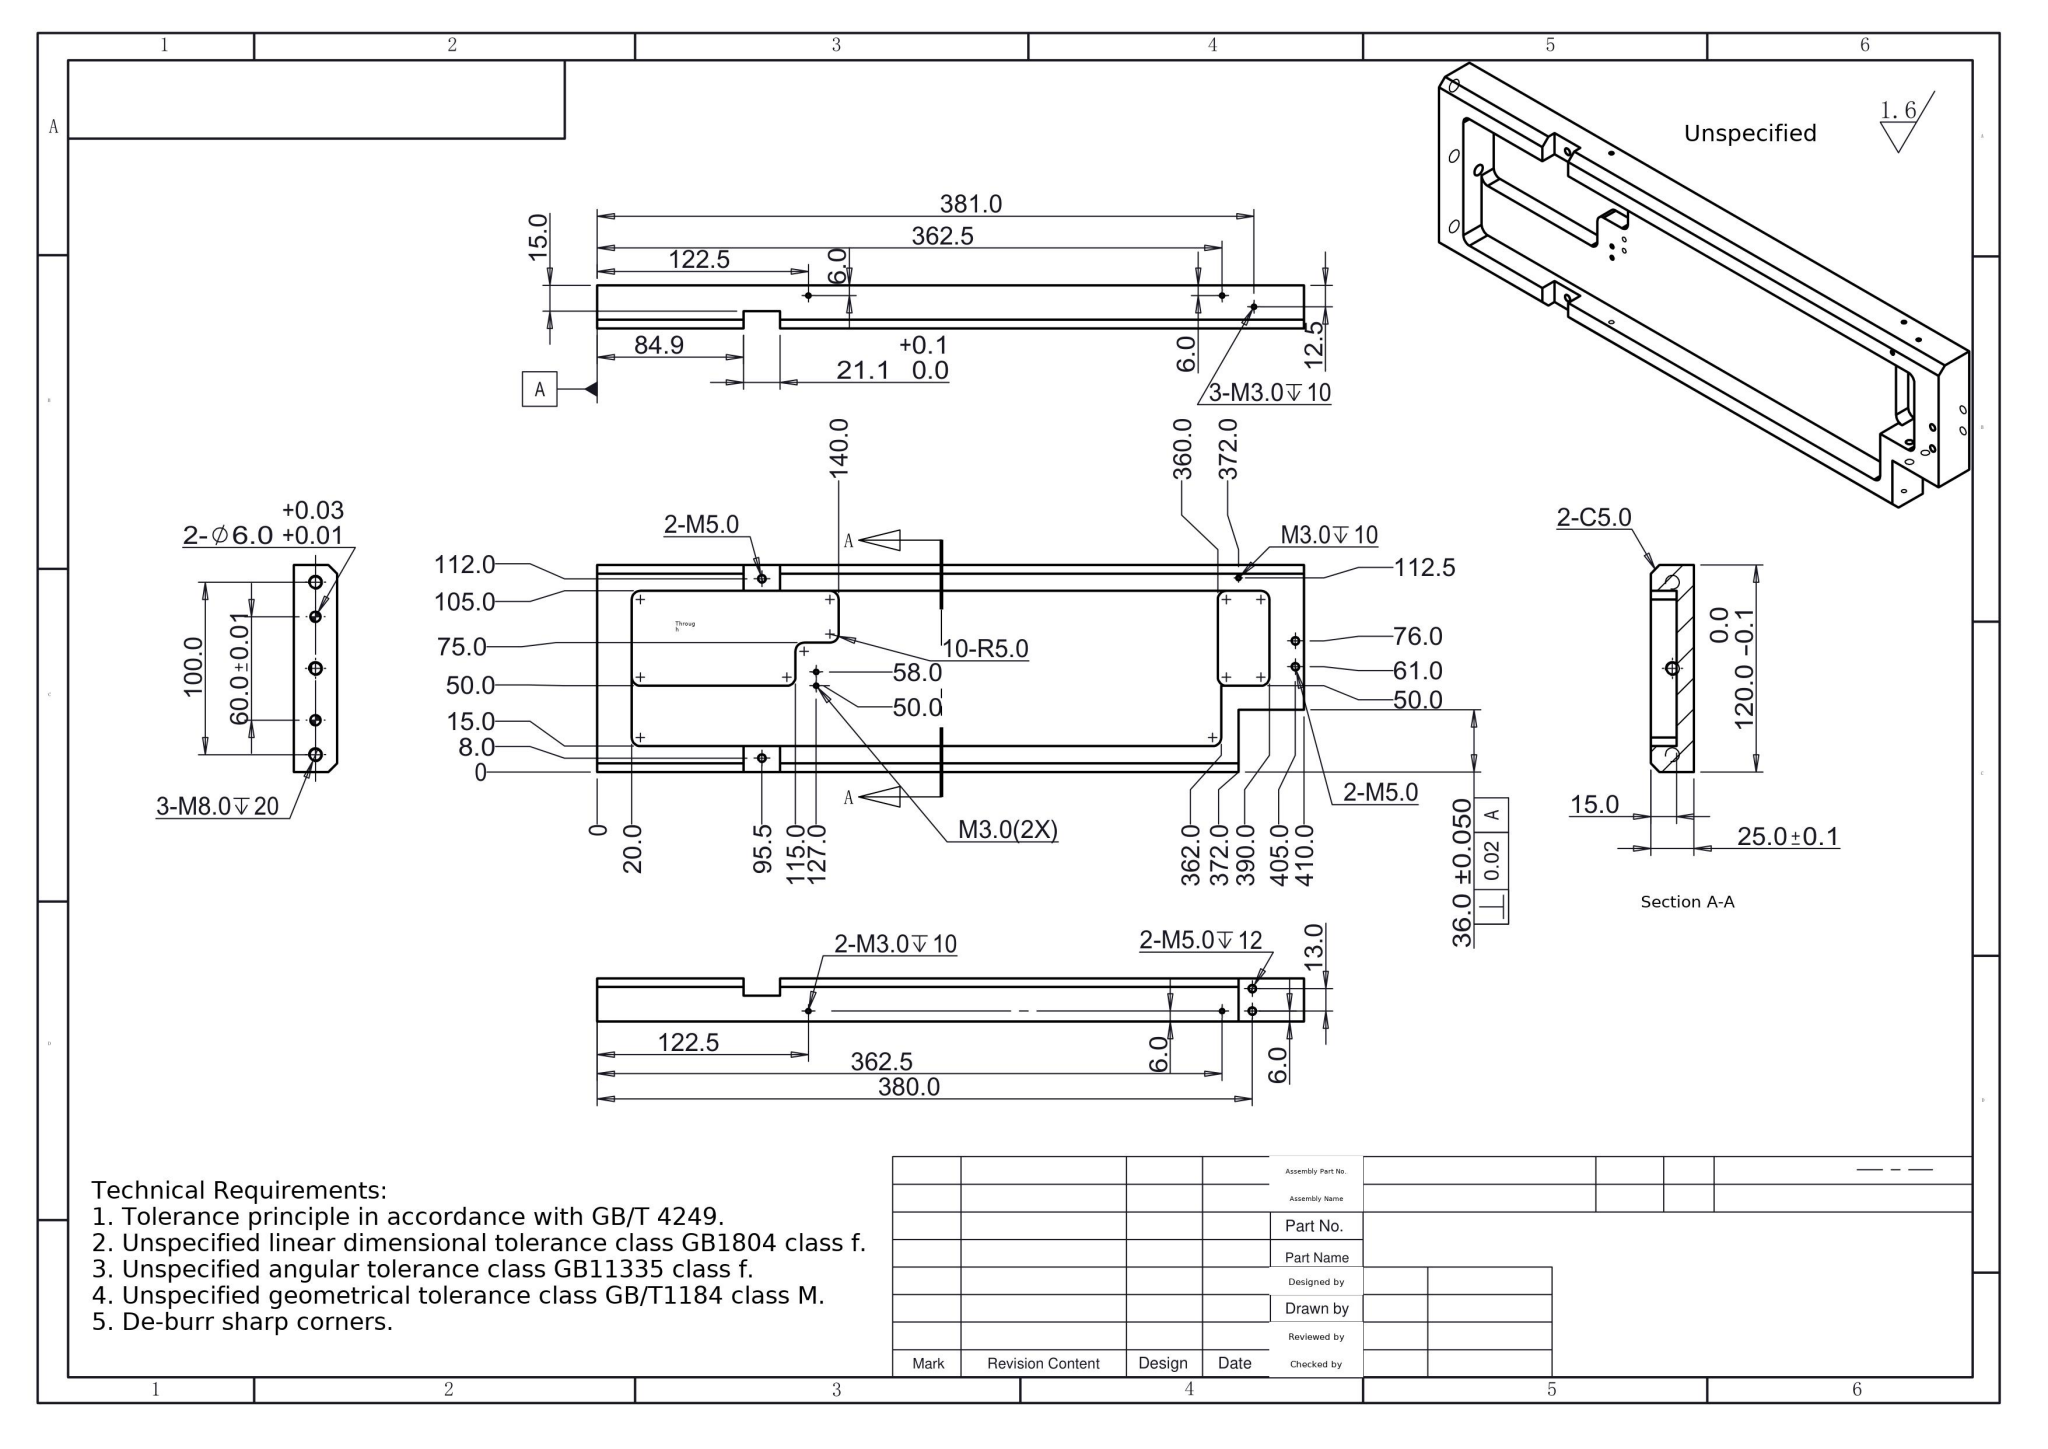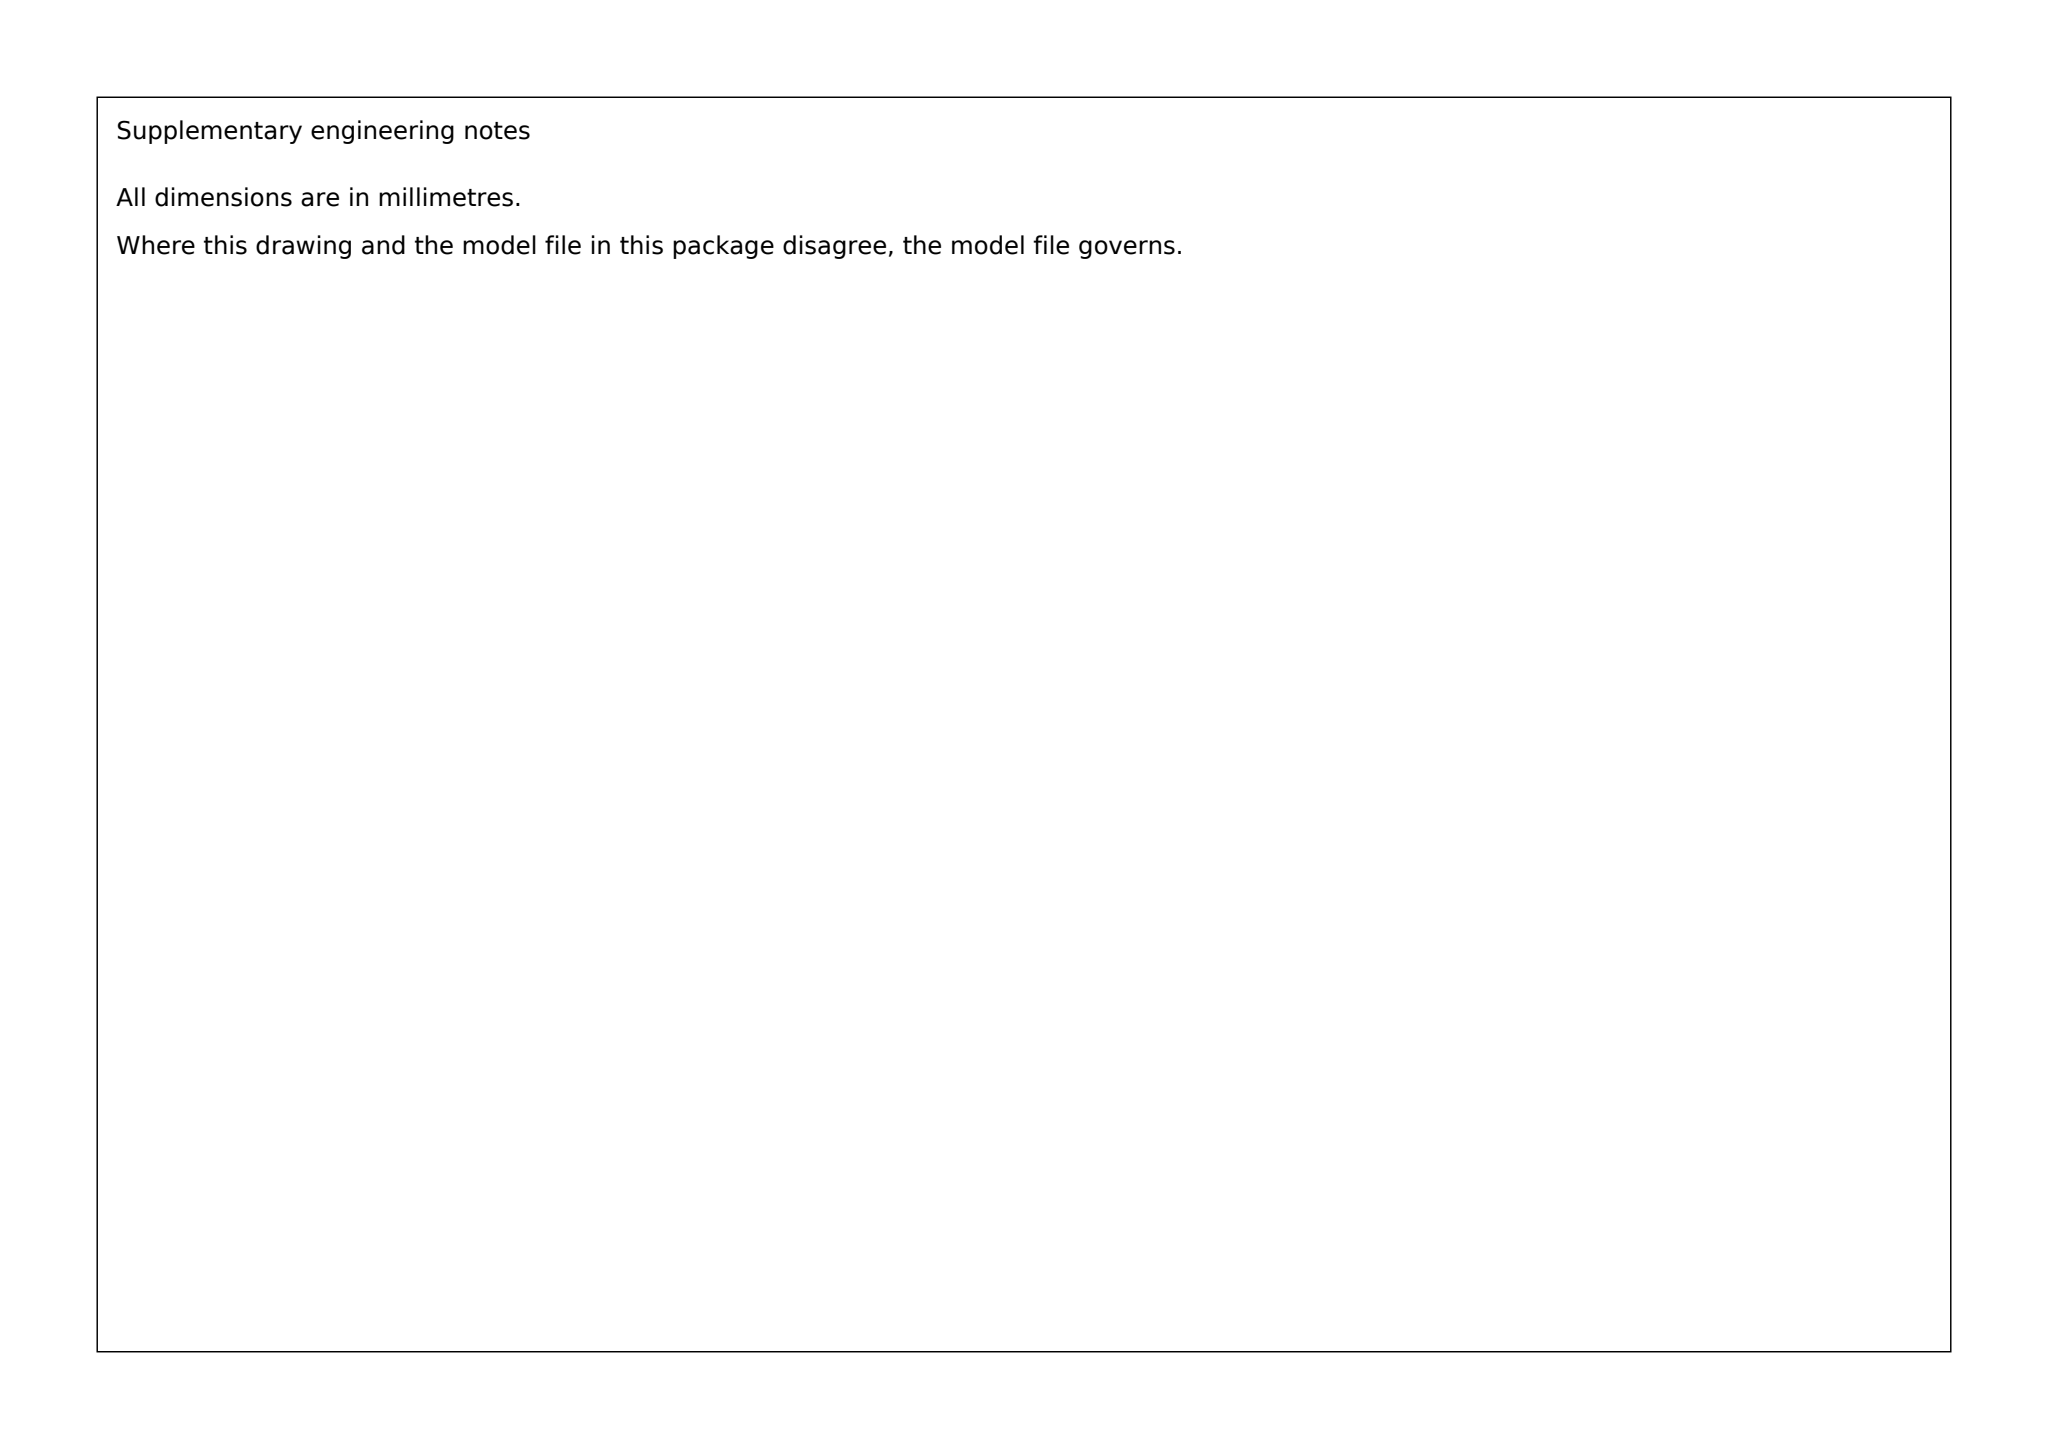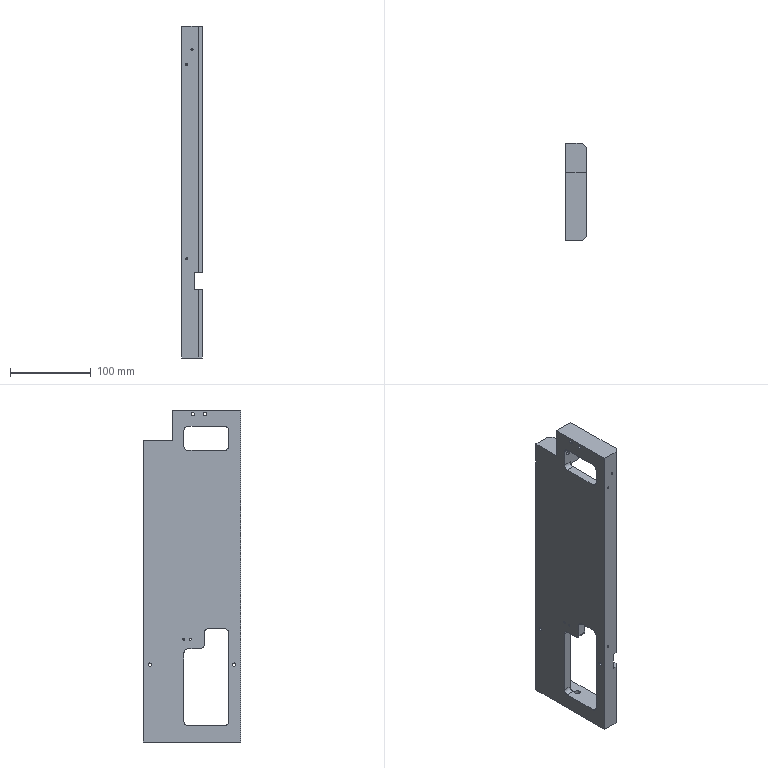Part | SolidWorks | mm | 1 solid | 101 faces | box 25 x 120 x 410 mm | volume 614983 mm3 | cylinder 50 | plane 31 | cone 20 | commonest cylinder face diameters 2.5 x16 4.2 x12 10 x12 6.8 x6 6 x4
build123d program:
from build123d import *

# Parameters (mm, degrees)
SKETCH1_W                    = 25
SKETCH1_H                    = 120
EXTRUDE1_DEPTH               = 205
M8_TAPPED_HOLE1_D            = 6.8
M8_TAPPED_HOLE1_DEPTH        = 23.75
M8_TAPPED_HOLE1_TIP          = 2.043
EXTRUDE2_DEPTH               = 15
EXTRUDE3_DEPTH               = 215.126
F_6_0_6_DIAMETER_HOLE1_D     = 6
F_6_0_6_DIAMETER_HOLE1_DEPTH = 10
F_6_0_6_DIAMETER_HOLE1_TIP   = 1.803
M3_TAPPED_HOLE1_AT_2_COUNT   = 2
M3_TAPPED_HOLE1_AT_2_PITCH   = 240
SKETCH18_W                   = 21.1
SKETCH18_H                   = 150.152
CUT_EXTRUDE1_DEPTH           = 10
M5_TAPPED_HOLE6_D            = 4.2
M5_TAPPED_HOLE6_DEPTH        = 17.4
M5_TAPPED_HOLE6_TIP          = 1.262
CHAMFER2_SIZE                = 5
SKETCH34_W                   = 99.744
SKETCH34_H                   = 340.807
CUT_EXTRUDE3_DEPTH           = 36
M5_TAPPED_HOLE7_D            = 4.2
M5_TAPPED_HOLE7_DEPTH        = 17.4
M5_TAPPED_HOLE7_TIP          = 1.262
M5_TAPPED_HOLE4_D            = 4.2
M5_TAPPED_HOLE4_DEPTH        = 32.4
M5_TAPPED_HOLE4_TIP          = 1.262
CUT_EXTRUDE4_REACH           = 217.058
M3_TAPPED_HOLE3_D            = 2.5
M3_TAPPED_HOLE3_DEPTH        = 9.5
M3_TAPPED_HOLE3_TIP          = 0.7511
M3_TAPPED_HOLE4_D            = 2.5
M3_TAPPED_HOLE4_DEPTH        = 9.5
M3_TAPPED_HOLE4_TIP          = 0.7511
SKETCH40_W                   = 25
SKETCH40_H                   = 25
BOSS_EXTRUDE1_DEPTH          = 10
FILLET1_R                    = 5
M3_TAPPED_HOLE5_D            = 2.5
M3_TAPPED_HOLE5_DEPTH        = 13.5
M3_TAPPED_HOLE5_TIP          = 0.7511


with BuildPart() as part:
    # Sketch1 → Extrude1 (new, symmetric)
    with BuildSketch(Plane.XY):
        Rectangle(SKETCH1_W, SKETCH1_H)
    extrude(amount=EXTRUDE1_DEPTH, both=True)

    # M8 Tapped Hole1
    with Locations(Plane(origin=(0, 0, -205), x_dir=(-1, 0, 0), z_dir=(0, 0, -1))):
        with Locations((0, 50), (0, -50), (0, 0)):
            Hole(M8_TAPPED_HOLE1_D / 2, depth=M8_TAPPED_HOLE1_DEPTH)
            with Locations((0, 0, -(M8_TAPPED_HOLE1_DEPTH + M8_TAPPED_HOLE1_TIP / 2))):  # 118° drill point
                Cone(0, M8_TAPPED_HOLE1_D / 2, M8_TAPPED_HOLE1_TIP, mode=Mode.SUBTRACT)

    # Sketch7 → Extrude2 (cut)
    with BuildSketch(Plane(origin=(12.5, 0, 0), x_dir=(0, 0, -1), z_dir=(1, 0, 0))):
        with BuildLine():
            Line((-180, 10), (180, 10))
            ThreePointArc((180, 10), (183.536, 8.536), (185, 5))
            Line((185, 5), (185, -40))
            ThreePointArc((185, -40), (183.536, -43.536), (180, -45))
            Line((180, -45), (-180, -45))
            ThreePointArc((-180, -45), (-183.536, -43.536), (-185, -40))
            Line((-185, -40), (-185, 5))
            ThreePointArc((-185, 5), (-183.536, 8.536), (-180, 10))
        make_face()
    extrude(amount=-EXTRUDE2_DEPTH, mode=Mode.SUBTRACT)

    # Sketch9 → Extrude3 (cut, through all)
    with BuildSketch(Plane(origin=(-2.5, 0, 0), x_dir=(0, 0, -1), z_dir=(1, 0, 0))):
        with BuildLine():
            Line((185, -40), (185, 5))
            ThreePointArc((185, 5), (183.536, 8.536), (180, 10))
            Line((180, 10), (70, 10))
            ThreePointArc((70, 10), (66.464, 8.536), (65, 5))
            Line((65, 5), (65, -40))
            ThreePointArc((65, -40), (66.464, -43.536), (70, -45))
            Line((70, -45), (180, -45))
            ThreePointArc((180, -45), (183.536, -43.536), (185, -40))
        make_face()
        with BuildLine():
            Line((-180, -45), (-160, -45))
            ThreePointArc((-160, -45), (-156.464, -43.536), (-155, -40))
            Line((-155, -40), (-155, 5))
            ThreePointArc((-155, 5), (-156.464, 8.536), (-160, 10))
            Line((-160, 10), (-180, 10))
            ThreePointArc((-180, 10), (-183.536, 8.536), (-185, 5))
            Line((-185, 5), (-185, -40))
            ThreePointArc((-185, -40), (-183.536, -43.536), (-180, -45))
        make_face()
    extrude(amount=-EXTRUDE3_DEPTH, mode=Mode.SUBTRACT)

    # 6.0 _6_ Diameter Hole1
    with Locations(Plane(origin=(0, 0, -205), x_dir=(-1, 0, 0), z_dir=(0, 0, -1))):
        with Locations((0, -30), (0, 30)):
            Hole(F_6_0_6_DIAMETER_HOLE1_D / 2, depth=F_6_0_6_DIAMETER_HOLE1_DEPTH)
            with Locations((0, 0, -(F_6_0_6_DIAMETER_HOLE1_DEPTH + F_6_0_6_DIAMETER_HOLE1_TIP / 2))):  # 118° drill point
                Cone(0, F_6_0_6_DIAMETER_HOLE1_D / 2, F_6_0_6_DIAMETER_HOLE1_TIP, mode=Mode.SUBTRACT)

    # Sketch16 → M3 Tapped Hole1 (revolve, cut)
    with BuildSketch(Plane(origin=(-6.5, -60, -82.5), x_dir=(0, 0, -1), z_dir=(1, 0, 0))):
        Polygon((0, 0), (0, 12.251), (1.25, 11.5), (1.25, 0), align=None)
    m3_tapped_hole1 = revolve(axis=Axis((-6.5, -66.35, -82.5), (0, 1, 0)), mode=Mode.SUBTRACT)

    # M3 Tapped Hole1 at 2: M3 Tapped Hole1 ×2
    with Locations(*[(0, 0, i * M3_TAPPED_HOLE1_AT_2_PITCH) for i in range(1, M3_TAPPED_HOLE1_AT_2_COUNT)]):
        add(m3_tapped_hole1, mode=Mode.SUBTRACT)

    # Mirror2: M3 Tapped Hole1 across plane
    add(m3_tapped_hole1.mirror(Plane.ZX), mode=Mode.SUBTRACT)

    # Mirror2 copy 1 sketch → Mirror2 copy 1 (revolve, cut)
    with BuildSketch(Plane(origin=(-6.5, 60, 157.5), x_dir=(0, 0, -1), z_dir=(1, 0, 0))):
        Polygon((0, 0), (0, -12.251), (1.25, -11.5), (1.25, 0), align=None)
    revolve(axis=Axis((-6.5, 66.35, 157.5), (0, 1, 0)), mode=Mode.SUBTRACT)

    # Sketch18 → Cut-Extrude1 (cut)
    with BuildSketch(Plane(origin=(12.5, 0, 0), x_dir=(0, 0, -1), z_dir=(1, 0, 0))):
        with Locations((109.55, 7.017)):
            Rectangle(SKETCH18_W, SKETCH18_H)
    extrude(amount=-CUT_EXTRUDE1_DEPTH, mode=Mode.SUBTRACT)

    # M5 Tapped Hole6
    with Locations(Plane(origin=(2.5, 0, 0), x_dir=(0, 0, -1), z_dir=(1, 0, 0))):
        with Locations((109.5, 52), (109.5, -52)):
            Hole(M5_TAPPED_HOLE6_D / 2, depth=M5_TAPPED_HOLE6_DEPTH)
            with Locations((0, 0, -(M5_TAPPED_HOLE6_DEPTH + M5_TAPPED_HOLE6_TIP / 2))):  # 118° drill point
                Cone(0, M5_TAPPED_HOLE6_D / 2, M5_TAPPED_HOLE6_TIP, mode=Mode.SUBTRACT)

    # Chamfer2
    chamfer2_edges = [part.edges().sort_by_distance(p)[0] for p in [
        (12.5, -60, -162.55),
        (12.5, 60, -162.55),
        (12.5, -60, 53),
        (12.5, 60, 53),
    ]]
    chamfer(chamfer2_edges, length=CHAMFER2_SIZE)

    # Sketch34 → Cut-Extrude3 (cut)
    with BuildSketch(Plane(origin=(0, 60, 0), x_dir=(1, 0, 0), z_dir=(0, 1, 0))):
        with Locations((-10.006, -337.403)):
            Rectangle(SKETCH34_W, SKETCH34_H)
    extrude(amount=-CUT_EXTRUDE3_DEPTH, mode=Mode.SUBTRACT)

    # M5 Tapped Hole7
    with Locations(Plane(origin=(-2.387, 24, 13.92), x_dir=(-1, 0, 0), z_dir=(0, 1, 0))):
        with Locations((-8.887, 161.08), (4.113, 161.08)):
            Hole(M5_TAPPED_HOLE7_D / 2, depth=M5_TAPPED_HOLE7_DEPTH)
            with Locations((0, 0, -(M5_TAPPED_HOLE7_DEPTH + M5_TAPPED_HOLE7_TIP / 2))):  # 118° drill point
                Cone(0, M5_TAPPED_HOLE7_D / 2, M5_TAPPED_HOLE7_TIP, mode=Mode.SUBTRACT)

    # M5 Tapped Hole4
    with Locations(Plane.ZY.offset(12.5)):
        with Locations((200, -16), (200, -1)):
            Hole(M5_TAPPED_HOLE4_D / 2, depth=M5_TAPPED_HOLE4_DEPTH)
            with Locations((0, 0, -(M5_TAPPED_HOLE4_DEPTH + M5_TAPPED_HOLE4_TIP / 2))):  # 118° drill point
                Cone(0, M5_TAPPED_HOLE4_D / 2, M5_TAPPED_HOLE4_TIP, mode=Mode.SUBTRACT)

    # Cut-Extrude4: up to this face of the body (flat: up to its plane)
    cut_extrude4_end = Plane(part.part.faces().sort_by_distance((-2.5, -17.5, 45))[0])
    # Sketch35 → Cut-Extrude4 (cut, up to the picked face)
    with BuildSketch(Plane(origin=(12.5, 0, 0), x_dir=(0, 0, -1), z_dir=(1, 0, 0)), mode=Mode.PRIVATE) as cut_extrude4_sk1:
        with BuildLine():
            Line((185, 5), (-157, 5))
            Line((-157, 5), (-157, 40))
            ThreePointArc((-157, 40), (-155.536, 43.536), (-152, 45))
            Line((-152, 45), (180, 45))
            ThreePointArc((180, 45), (183.536, 43.536), (185, 40))
            Line((185, 40), (185, 5))
        make_face()
    cut_extrude4_tool1 = split(extrude(cut_extrude4_sk1.sketch, amount=-CUT_EXTRUDE4_REACH, mode=Mode.PRIVATE), bisect_by=cut_extrude4_end, keep=Keep.BOTH, mode=Mode.PRIVATE)
    add(cut_extrude4_tool1.solids().sort_by(Axis((12.5, 24.985, -14), (-1, 0, 0)))[0], mode=Mode.SUBTRACT)

    # M3 Tapped Hole3
    with Locations(Plane(origin=(12.5, 0, 0), x_dir=(0, 0, -1), z_dir=(1, 0, 0))):
        with Locations((-167, -52.5)):
            Hole(M3_TAPPED_HOLE3_D / 2, depth=M3_TAPPED_HOLE3_DEPTH)
            with Locations((0, 0, -(M3_TAPPED_HOLE3_DEPTH + M3_TAPPED_HOLE3_TIP / 2))):  # 118° drill point
                Cone(0, M3_TAPPED_HOLE3_D / 2, M3_TAPPED_HOLE3_TIP, mode=Mode.SUBTRACT)

    # M3 Tapped Hole4
    with Locations(Plane.XZ.offset(60)):
        with Locations((0, 176)):
            Hole(M3_TAPPED_HOLE4_D / 2, depth=M3_TAPPED_HOLE4_DEPTH)
            with Locations((0, 0, -(M3_TAPPED_HOLE4_DEPTH + M3_TAPPED_HOLE4_TIP / 2))):  # 118° drill point
                Cone(0, M3_TAPPED_HOLE4_D / 2, M3_TAPPED_HOLE4_TIP, mode=Mode.SUBTRACT)

    # Sketch40 → Boss-Extrude1 (add)
    with BuildSketch(Plane.ZY.offset(12.5)):
        with Locations((-77.5, -2.5)):
            Rectangle(SKETCH40_W, SKETCH40_H)
    extrude(amount=-BOSS_EXTRUDE1_DEPTH)

    # Fillet1
    fillet1_edges = [part.edges().sort_by_distance(p)[0] for p in [
        (-7.5, 10, -90),
        (-7.5, -15, -90),
        (-7.5, -15, -65),
    ]]
    fillet(fillet1_edges, radius=FILLET1_R)

    # M3 Tapped Hole5
    with Locations(Plane.ZY.offset(12.5)):
        with Locations((-78, 2), (-78, 10)):
            Hole(M3_TAPPED_HOLE5_D / 2, depth=M3_TAPPED_HOLE5_DEPTH)
            with Locations((0, 0, -(M3_TAPPED_HOLE5_DEPTH + M3_TAPPED_HOLE5_TIP / 2))):  # 118° drill point
                Cone(0, M3_TAPPED_HOLE5_D / 2, M3_TAPPED_HOLE5_TIP, mode=Mode.SUBTRACT)


solid = part.part